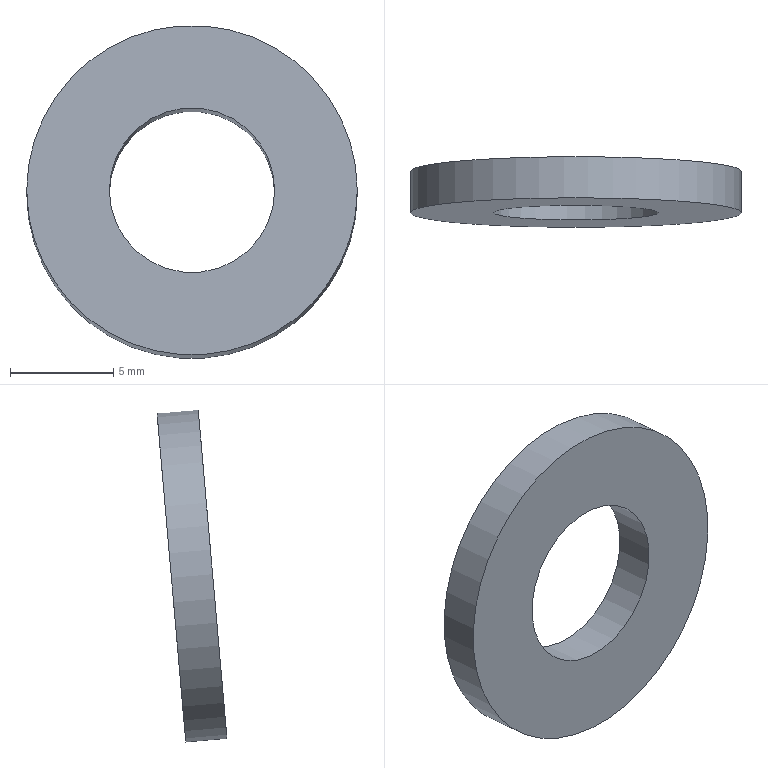Component | NX | SMALL_WASHER | 1 solid | 4 faces | box 16 x 3.39 x 16.11 mm | volume 302 mm3 | cylinder 2 | plane 2 | commonest cylinder face diameters 16 x1 8 x1
STEP:
#1=CARTESIAN_POINT('',(0.,0.,0.));
#2=DIRECTION('',(0.,0.,1.));
#3=DIRECTION('',(1.,0.,0.));
#4=AXIS2_PLACEMENT_3D('',#1,#2,#3);
#5=CARTESIAN_POINT('',(283.941,462.114,-25.155));
#6=VERTEX_POINT('',#5);
#7=CARTESIAN_POINT('',(275.941,462.114,-25.155));
#8=DIRECTION('',(0.,-0.9962,0.08716));
#9=DIRECTION('',(1.,0.,0.));
#10=AXIS2_PLACEMENT_3D('',#7,#8,#9);
#11=CIRCLE('',#10,8.);
#12=CARTESIAN_POINT('',(275.941,462.114,-25.155));
#13=DIRECTION('',(0.,0.9962,-0.08716));
#14=DIRECTION('',(-1.,0.,0.));
#15=AXIS2_PLACEMENT_3D('',#12,#13,#14);
#16=CYLINDRICAL_SURFACE('',#15,8.);
#17=CARTESIAN_POINT('',(9.425,0.));
#18=DIRECTION('',(-1.,0.));
#19=VECTOR('',#18,1.);
#20=LINE('',#17,#19);
#21=(GEOMETRIC_REPRESENTATION_CONTEXT(2)PARAMETRIC_REPRESENTATION_CONTEXT()REPRESENTATION_CONTEXT('',''));
#22=DEFINITIONAL_REPRESENTATION('',(#20),#21);
#23=PCURVE('',#16,#22);
#24=CARTESIAN_POINT('',(275.941,462.114,-25.155));
#25=DIRECTION('',(0.,-0.9962,0.08716));
#26=DIRECTION('',(1.,0.,0.));
#27=AXIS2_PLACEMENT_3D('',#24,#25,#26);
#28=PLANE('',#27);
#29=CARTESIAN_POINT('',(0.,0.));
#30=DIRECTION('',(1.,0.));
#31=AXIS2_PLACEMENT_2D('',#29,#30);
#32=CIRCLE('',#31,8.);
#33=(GEOMETRIC_REPRESENTATION_CONTEXT(2)PARAMETRIC_REPRESENTATION_CONTEXT()REPRESENTATION_CONTEXT('',''));
#34=DEFINITIONAL_REPRESENTATION('',(#32),#33);
#35=PCURVE('',#28,#34);
#36=SURFACE_CURVE('',#11,(#23,#35),.PCURVE_S1.);
#37=EDGE_CURVE('',#6,#6,#36,.T.);
#38=ORIENTED_EDGE('',*,*,#37,.F.);
#39=CARTESIAN_POINT('',(283.941,464.106,-25.33));
#40=VERTEX_POINT('',#39);
#41=CARTESIAN_POINT('',(283.941,462.114,-25.155));
#42=CARTESIAN_POINT('',(283.941,464.106,-25.33));
#43=B_SPLINE_CURVE_WITH_KNOTS('',1,(#41,#42),.UNSPECIFIED.,.F.,.F.,(2,2),(0.,2.),.PIECEWISE_BEZIER_KNOTS.);
#44=CARTESIAN_POINT('',(9.425,0.));
#45=DIRECTION('',(0.,1.));
#46=VECTOR('',#45,1.);
#47=LINE('',#44,#46);
#48=(GEOMETRIC_REPRESENTATION_CONTEXT(2)PARAMETRIC_REPRESENTATION_CONTEXT()REPRESENTATION_CONTEXT('',''));
#49=DEFINITIONAL_REPRESENTATION('',(#47),#48);
#50=PCURVE('',#16,#49);
#51=CARTESIAN_POINT('',(3.142,0.));
#52=DIRECTION('',(0.,1.));
#53=VECTOR('',#52,1.);
#54=LINE('',#51,#53);
#55=(GEOMETRIC_REPRESENTATION_CONTEXT(2)PARAMETRIC_REPRESENTATION_CONTEXT()REPRESENTATION_CONTEXT('',''));
#56=DEFINITIONAL_REPRESENTATION('',(#54),#55);
#57=PCURVE('',#16,#56);
#58=SEAM_CURVE('',#43,(#50,#57),.PCURVE_S1.);
#59=EDGE_CURVE('',#6,#40,#58,.T.);
#60=ORIENTED_EDGE('',*,*,#59,.T.);
#61=CARTESIAN_POINT('',(275.941,464.106,-25.33));
#62=DIRECTION('',(0.,-0.9962,0.08716));
#63=DIRECTION('',(1.,0.,0.));
#64=AXIS2_PLACEMENT_3D('',#61,#62,#63);
#65=CIRCLE('',#64,8.);
#66=CARTESIAN_POINT('',(9.425,2.));
#67=DIRECTION('',(-1.,0.));
#68=VECTOR('',#67,1.);
#69=LINE('',#66,#68);
#70=(GEOMETRIC_REPRESENTATION_CONTEXT(2)PARAMETRIC_REPRESENTATION_CONTEXT()REPRESENTATION_CONTEXT('',''));
#71=DEFINITIONAL_REPRESENTATION('',(#69),#70);
#72=PCURVE('',#16,#71);
#73=CARTESIAN_POINT('',(275.941,464.106,-25.33));
#74=DIRECTION('',(0.,-0.9962,0.08716));
#75=DIRECTION('',(1.,0.,0.));
#76=AXIS2_PLACEMENT_3D('',#73,#74,#75);
#77=PLANE('',#76);
#78=CARTESIAN_POINT('',(0.,0.));
#79=DIRECTION('',(1.,0.));
#80=AXIS2_PLACEMENT_2D('',#78,#79);
#81=CIRCLE('',#80,8.);
#82=(GEOMETRIC_REPRESENTATION_CONTEXT(2)PARAMETRIC_REPRESENTATION_CONTEXT()REPRESENTATION_CONTEXT('',''));
#83=DEFINITIONAL_REPRESENTATION('',(#81),#82);
#84=PCURVE('',#77,#83);
#85=SURFACE_CURVE('',#65,(#72,#84),.PCURVE_S1.);
#86=EDGE_CURVE('',#40,#40,#85,.T.);
#87=ORIENTED_EDGE('',*,*,#86,.T.);
#88=ORIENTED_EDGE('',*,*,#59,.F.);
#89=EDGE_LOOP('',(#38,#60,#87,#88));
#90=FACE_BOUND('',#89,.T.);
#91=ADVANCED_FACE('',(#90),#16,.T.);
#92=CARTESIAN_POINT('',(279.941,462.114,-25.155));
#93=VERTEX_POINT('',#92);
#94=CARTESIAN_POINT('',(275.941,462.114,-25.155));
#95=DIRECTION('',(0.,-0.9962,0.08716));
#96=DIRECTION('',(1.,0.,0.));
#97=AXIS2_PLACEMENT_3D('',#94,#95,#96);
#98=CIRCLE('',#97,4.);
#99=CARTESIAN_POINT('',(275.941,462.114,-25.155));
#100=DIRECTION('',(0.,0.9962,-0.08716));
#101=DIRECTION('',(-1.,0.,0.));
#102=AXIS2_PLACEMENT_3D('',#99,#100,#101);
#103=CYLINDRICAL_SURFACE('',#102,4.);
#104=CARTESIAN_POINT('',(9.425,0.));
#105=DIRECTION('',(-1.,0.));
#106=VECTOR('',#105,1.);
#107=LINE('',#104,#106);
#108=(GEOMETRIC_REPRESENTATION_CONTEXT(2)PARAMETRIC_REPRESENTATION_CONTEXT()REPRESENTATION_CONTEXT('',''));
#109=DEFINITIONAL_REPRESENTATION('',(#107),#108);
#110=PCURVE('',#103,#109);
#111=CARTESIAN_POINT('',(0.,0.));
#112=DIRECTION('',(1.,0.));
#113=AXIS2_PLACEMENT_2D('',#111,#112);
#114=CIRCLE('',#113,4.);
#115=(GEOMETRIC_REPRESENTATION_CONTEXT(2)PARAMETRIC_REPRESENTATION_CONTEXT()REPRESENTATION_CONTEXT('',''));
#116=DEFINITIONAL_REPRESENTATION('',(#114),#115);
#117=PCURVE('',#28,#116);
#118=SURFACE_CURVE('',#98,(#110,#117),.PCURVE_S1.);
#119=EDGE_CURVE('',#93,#93,#118,.T.);
#120=ORIENTED_EDGE('',*,*,#119,.F.);
#121=CARTESIAN_POINT('',(279.941,464.106,-25.33));
#122=VERTEX_POINT('',#121);
#123=CARTESIAN_POINT('',(279.941,462.114,-25.155));
#124=CARTESIAN_POINT('',(279.941,464.106,-25.33));
#125=B_SPLINE_CURVE_WITH_KNOTS('',1,(#123,#124),.UNSPECIFIED.,.F.,.F.,(2,2),(0.,2.),.PIECEWISE_BEZIER_KNOTS.);
#126=CARTESIAN_POINT('',(9.425,0.));
#127=DIRECTION('',(0.,1.));
#128=VECTOR('',#127,1.);
#129=LINE('',#126,#128);
#130=(GEOMETRIC_REPRESENTATION_CONTEXT(2)PARAMETRIC_REPRESENTATION_CONTEXT()REPRESENTATION_CONTEXT('',''));
#131=DEFINITIONAL_REPRESENTATION('',(#129),#130);
#132=PCURVE('',#103,#131);
#133=CARTESIAN_POINT('',(3.142,0.));
#134=DIRECTION('',(0.,1.));
#135=VECTOR('',#134,1.);
#136=LINE('',#133,#135);
#137=(GEOMETRIC_REPRESENTATION_CONTEXT(2)PARAMETRIC_REPRESENTATION_CONTEXT()REPRESENTATION_CONTEXT('',''));
#138=DEFINITIONAL_REPRESENTATION('',(#136),#137);
#139=PCURVE('',#103,#138);
#140=SEAM_CURVE('',#125,(#132,#139),.PCURVE_S1.);
#141=EDGE_CURVE('',#93,#122,#140,.T.);
#142=ORIENTED_EDGE('',*,*,#141,.T.);
#143=CARTESIAN_POINT('',(275.941,464.106,-25.33));
#144=DIRECTION('',(0.,-0.9962,0.08716));
#145=DIRECTION('',(1.,0.,0.));
#146=AXIS2_PLACEMENT_3D('',#143,#144,#145);
#147=CIRCLE('',#146,4.);
#148=CARTESIAN_POINT('',(9.425,2.));
#149=DIRECTION('',(-1.,0.));
#150=VECTOR('',#149,1.);
#151=LINE('',#148,#150);
#152=(GEOMETRIC_REPRESENTATION_CONTEXT(2)PARAMETRIC_REPRESENTATION_CONTEXT()REPRESENTATION_CONTEXT('',''));
#153=DEFINITIONAL_REPRESENTATION('',(#151),#152);
#154=PCURVE('',#103,#153);
#155=CARTESIAN_POINT('',(0.,0.));
#156=DIRECTION('',(1.,0.));
#157=AXIS2_PLACEMENT_2D('',#155,#156);
#158=CIRCLE('',#157,4.);
#159=(GEOMETRIC_REPRESENTATION_CONTEXT(2)PARAMETRIC_REPRESENTATION_CONTEXT()REPRESENTATION_CONTEXT('',''));
#160=DEFINITIONAL_REPRESENTATION('',(#158),#159);
#161=PCURVE('',#77,#160);
#162=SURFACE_CURVE('',#147,(#154,#161),.PCURVE_S1.);
#163=EDGE_CURVE('',#122,#122,#162,.T.);
#164=ORIENTED_EDGE('',*,*,#163,.T.);
#165=ORIENTED_EDGE('',*,*,#141,.F.);
#166=EDGE_LOOP('',(#120,#142,#164,#165));
#167=FACE_BOUND('',#166,.F.);
#168=ADVANCED_FACE('',(#167),#103,.F.);
#169=ORIENTED_EDGE('',*,*,#37,.T.);
#170=EDGE_LOOP('',(#169));
#171=FACE_BOUND('',#170,.T.);
#172=ORIENTED_EDGE('',*,*,#119,.F.);
#173=EDGE_LOOP('',(#172));
#174=FACE_BOUND('',#173,.T.);
#175=ADVANCED_FACE('',(#171,#174),#28,.T.);
#176=ORIENTED_EDGE('',*,*,#86,.F.);
#177=EDGE_LOOP('',(#176));
#178=FACE_BOUND('',#177,.T.);
#179=ORIENTED_EDGE('',*,*,#163,.T.);
#180=EDGE_LOOP('',(#179));
#181=FACE_BOUND('',#180,.T.);
#182=ADVANCED_FACE('',(#178,#181),#77,.F.);
#183=CLOSED_SHELL('',(#91,#168,#175,#182));
#184=MANIFOLD_SOLID_BREP('',#183);
#185=(LENGTH_UNIT()NAMED_UNIT(*)SI_UNIT(.MILLI.,.METRE.));
#186=UNCERTAINTY_MEASURE_WITH_UNIT(LENGTH_MEASURE(0.00001),#185,'','');
#187=(NAMED_UNIT(*)PLANE_ANGLE_UNIT()SI_UNIT($,.RADIAN.));
#188=(NAMED_UNIT(*)SI_UNIT($,.STERADIAN.)SOLID_ANGLE_UNIT());
#189=(GEOMETRIC_REPRESENTATION_CONTEXT(3)GLOBAL_UNCERTAINTY_ASSIGNED_CONTEXT((#186))GLOBAL_UNIT_ASSIGNED_CONTEXT((#185,#187,#188))REPRESENTATION_CONTEXT('',''));
#190=ADVANCED_BREP_SHAPE_REPRESENTATION('',(#4,#184),#189);